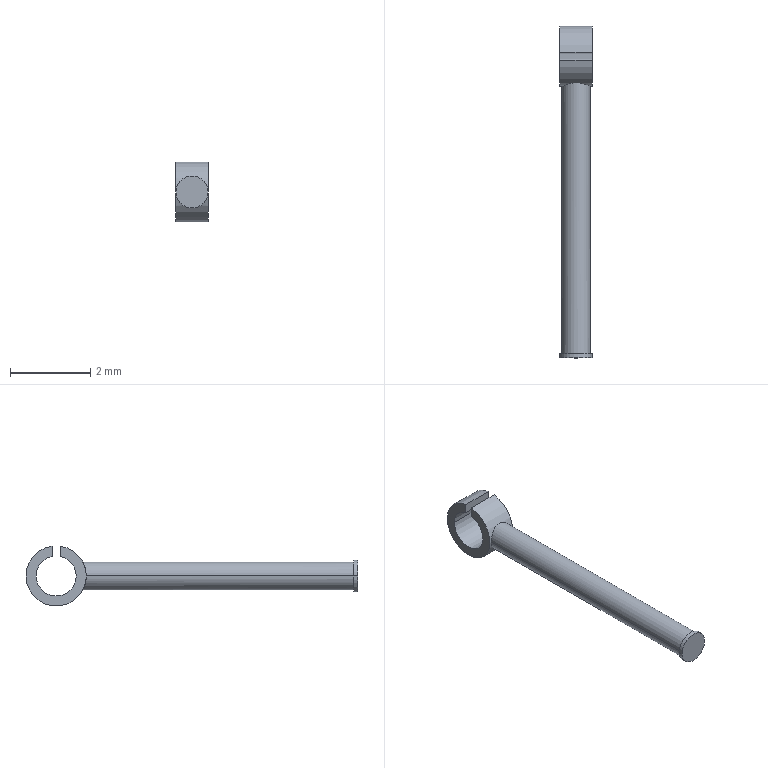Component | SolidWorks | PushRod-15 | 1 solid | 16 faces | box 0.8 x 8.26 x 1.49 mm | volume 3 mm3 | cylinder 10 | plane 6 | commonest cylinder face diameters 1 x3 1.5 x3 0.8 x2 0.7 x2
build123d program:
from build123d import *

# Parameters (mm, degrees)
BOSS_EXTRUDE1_DEPTH      = 3.75
BOSS_EXTRUDE1_DEPTH_BACK = 3
SKETCH2_R                = 0.35
SKETCH3_R                = 0.75
SKETCH3_R_2              = 0.5
BOSS_EXTRUDE2_DEPTH      = 0.4
SKETCH4_R                = 0.4
BOSS_EXTRUDE3_DEPTH      = 0.1
SKETCH5_W                = 0.2
SKETCH5_H                = 0.7342
CUT_EXTRUDE1_DEPTH       = 1


with BuildPart() as part:
    # Sketch2 → Boss-Extrude1 (new, two sides: drawn at the far end of the back side and taken through both)
    with BuildSketch(Plane.XY.offset(-BOSS_EXTRUDE1_DEPTH_BACK)):
        with Locations((-0.5, 1.5)):
            Circle(SKETCH2_R)
    extrude(amount=BOSS_EXTRUDE1_DEPTH + BOSS_EXTRUDE1_DEPTH_BACK)

    # Sketch3 → Boss-Extrude2 (add, symmetric)
    with BuildSketch(Plane(origin=(-0.5, 0, 0), x_dir=(0, 0, -1), z_dir=(1, 0, 0))):
        with Locations((-4.413, 1.5)):
            Circle(SKETCH3_R)
        with Locations((-4.413, 1.5)):
            Circle(SKETCH3_R_2, mode=Mode.SUBTRACT)
    extrude(amount=BOSS_EXTRUDE2_DEPTH, both=True)

    # Sketch4 → Boss-Extrude3 (add)
    with BuildSketch(Plane(origin=(0, 0, -3), x_dir=(-1, 0, 0), z_dir=(0, 0, -1))):
        with Locations((0.5, 1.5)):
            Circle(SKETCH4_R)
    extrude(amount=BOSS_EXTRUDE3_DEPTH)

    # Sketch5 → Cut-Extrude1 (cut)
    with BuildSketch(Plane(origin=(-0.1, 0, 0), x_dir=(0, 0, -1), z_dir=(1, 0, 0))):
        with Locations((-4.413, 0.75)):
            Rectangle(SKETCH5_W, SKETCH5_H)
    extrude(amount=-CUT_EXTRUDE1_DEPTH, mode=Mode.SUBTRACT)


solid = part.part

# Placed as in the assembly
solid = solid.moved(Location((10.347, 3.138, 9), (-90, 0, 0)))
STEP:
#1=COLOUR_RGB('',0.7922,0.8196,0.9333);
#2=FILL_AREA_STYLE_COLOUR('',#1);
#3=FILL_AREA_STYLE('',(#2));
#4=SURFACE_STYLE_FILL_AREA(#3);
#5=SURFACE_SIDE_STYLE('',(#4));
#6=SURFACE_STYLE_USAGE(.BOTH.,#5);
#7=PRESENTATION_STYLE_ASSIGNMENT((#6));
#8=CARTESIAN_POINT('',(0.3719,0.001518,0.2953));
#9=VERTEX_POINT('',#8);
#10=CARTESIAN_POINT('',(0.4034,0.001518,0.2953));
#11=VERTEX_POINT('',#10);
#12=CARTESIAN_POINT('',(0.3877,0.001518,0.2953));
#13=DIRECTION('',(0.,-1.,0.));
#14=DIRECTION('',(-1.,-0.,0.));
#15=AXIS2_PLACEMENT_3D('',#12,#13,#14);
#16=CIRCLE('',#15,0.01575);
#17=EDGE_CURVE('',#9,#11,#16,.T.);
#18=ORIENTED_EDGE('',*,*,#17,.F.);
#19=CARTESIAN_POINT('',(0.3719,0.005455,0.2953));
#20=VERTEX_POINT('',#19);
#21=CARTESIAN_POINT('',(0.3719,0.001518,0.2953));
#22=DIRECTION('',(-0.,1.,-0.));
#23=VECTOR('',#22,39.37);
#24=LINE('',#21,#23);
#25=EDGE_CURVE('',#9,#20,#24,.T.);
#26=ORIENTED_EDGE('',*,*,#25,.T.);
#27=CARTESIAN_POINT('',(0.4034,0.005455,0.2953));
#28=VERTEX_POINT('',#27);
#29=CARTESIAN_POINT('',(0.3877,0.005455,0.2953));
#30=DIRECTION('',(0.,-1.,0.));
#31=DIRECTION('',(-1.,-0.,0.));
#32=AXIS2_PLACEMENT_3D('',#29,#30,#31);
#33=CIRCLE('',#32,0.01575);
#34=EDGE_CURVE('',#20,#28,#33,.T.);
#35=ORIENTED_EDGE('',*,*,#34,.T.);
#36=CARTESIAN_POINT('',(0.4034,0.001518,0.2953));
#37=DIRECTION('',(-0.,1.,-0.));
#38=VECTOR('',#37,39.37);
#39=LINE('',#36,#38);
#40=EDGE_CURVE('',#11,#28,#39,.T.);
#41=ORIENTED_EDGE('',*,*,#40,.F.);
#42=EDGE_LOOP('',(#18,#26,#35,#41));
#43=FACE_OUTER_BOUND('',#42,.T.);
#44=CARTESIAN_POINT('',(0.3877,0.001518,0.2953));
#45=DIRECTION('',(-0.,1.,-0.));
#46=DIRECTION('',(1.,0.,0.));
#47=AXIS2_PLACEMENT_3D('',#44,#45,#46);
#48=CYLINDRICAL_SURFACE('',#47,0.01575);
#49=ADVANCED_FACE('',(#43),#48,.T.);
#50=CARTESIAN_POINT('',(0.4034,0.2934,0.3146));
#51=VERTEX_POINT('',#50);
#52=CARTESIAN_POINT('',(0.4034,0.2776,0.2953));
#53=VERTEX_POINT('',#52);
#54=CARTESIAN_POINT('',(0.4034,0.2973,0.2953));
#55=DIRECTION('',(1.,0.,0.));
#56=DIRECTION('',(0.,-1.,0.));
#57=AXIS2_PLACEMENT_3D('',#54,#55,#56);
#58=CIRCLE('',#57,0.01969);
#59=EDGE_CURVE('',#51,#53,#58,.T.);
#60=ORIENTED_EDGE('',*,*,#59,.T.);
#61=CARTESIAN_POINT('',(0.3719,0.2776,0.2953));
#62=VERTEX_POINT('',#61);
#63=CARTESIAN_POINT('',(0.4034,0.2776,0.2953));
#64=DIRECTION('',(-1.,-0.,0.));
#65=VECTOR('',#64,39.37);
#66=LINE('',#63,#65);
#67=EDGE_CURVE('',#53,#62,#66,.T.);
#68=ORIENTED_EDGE('',*,*,#67,.T.);
#69=CARTESIAN_POINT('',(0.3719,0.2934,0.3146));
#70=VERTEX_POINT('',#69);
#71=CARTESIAN_POINT('',(0.3719,0.2973,0.2953));
#72=DIRECTION('',(1.,0.,0.));
#73=DIRECTION('',(0.,-1.,0.));
#74=AXIS2_PLACEMENT_3D('',#71,#72,#73);
#75=CIRCLE('',#74,0.01969);
#76=EDGE_CURVE('',#70,#62,#75,.T.);
#77=ORIENTED_EDGE('',*,*,#76,.F.);
#78=CARTESIAN_POINT('',(0.4034,0.2934,0.3146));
#79=DIRECTION('',(-1.,-0.,0.));
#80=VECTOR('',#79,39.37);
#81=LINE('',#78,#80);
#82=EDGE_CURVE('',#51,#70,#81,.T.);
#83=ORIENTED_EDGE('',*,*,#82,.F.);
#84=EDGE_LOOP('',(#60,#68,#77,#83));
#85=FACE_OUTER_BOUND('',#84,.T.);
#86=CARTESIAN_POINT('',(0.4034,0.2973,0.2953));
#87=DIRECTION('',(-1.,-0.,0.));
#88=DIRECTION('',(0.,1.,0.));
#89=AXIS2_PLACEMENT_3D('',#86,#87,#88);
#90=CYLINDRICAL_SURFACE('',#89,0.01969);
#91=ADVANCED_FACE('',(#85),#90,.F.);
#92=ORIENTED_EDGE('',*,*,#67,.F.);
#93=CARTESIAN_POINT('',(0.4034,0.317,0.2953));
#94=VERTEX_POINT('',#93);
#95=CARTESIAN_POINT('',(0.4034,0.2973,0.2953));
#96=DIRECTION('',(1.,0.,0.));
#97=DIRECTION('',(0.,-1.,0.));
#98=AXIS2_PLACEMENT_3D('',#95,#96,#97);
#99=CIRCLE('',#98,0.01969);
#100=EDGE_CURVE('',#53,#94,#99,.T.);
#101=ORIENTED_EDGE('',*,*,#100,.T.);
#102=CARTESIAN_POINT('',(0.3719,0.317,0.2953));
#103=VERTEX_POINT('',#102);
#104=CARTESIAN_POINT('',(0.4034,0.317,0.2953));
#105=DIRECTION('',(-1.,-0.,0.));
#106=VECTOR('',#105,39.37);
#107=LINE('',#104,#106);
#108=EDGE_CURVE('',#94,#103,#107,.T.);
#109=ORIENTED_EDGE('',*,*,#108,.T.);
#110=CARTESIAN_POINT('',(0.3719,0.2973,0.2953));
#111=DIRECTION('',(1.,0.,0.));
#112=DIRECTION('',(0.,-1.,0.));
#113=AXIS2_PLACEMENT_3D('',#110,#111,#112);
#114=CIRCLE('',#113,0.01969);
#115=EDGE_CURVE('',#62,#103,#114,.T.);
#116=ORIENTED_EDGE('',*,*,#115,.F.);
#117=EDGE_LOOP('',(#92,#101,#109,#116));
#118=FACE_OUTER_BOUND('',#117,.T.);
#119=CARTESIAN_POINT('',(0.4034,0.2973,0.2953));
#120=DIRECTION('',(-1.,-0.,0.));
#121=DIRECTION('',(0.,1.,0.));
#122=AXIS2_PLACEMENT_3D('',#119,#120,#121);
#123=CYLINDRICAL_SURFACE('',#122,0.01969);
#124=ADVANCED_FACE('',(#118),#123,.F.);
#125=CARTESIAN_POINT('',(0.4034,0.2678,0.2953));
#126=VERTEX_POINT('',#125);
#127=CARTESIAN_POINT('',(0.4034,0.3268,0.2953));
#128=VERTEX_POINT('',#127);
#129=CARTESIAN_POINT('',(0.4034,0.2973,0.2953));
#130=DIRECTION('',(1.,0.,0.));
#131=DIRECTION('',(0.,-1.,0.));
#132=AXIS2_PLACEMENT_3D('',#129,#130,#131);
#133=CIRCLE('',#132,0.02953);
#134=EDGE_CURVE('',#126,#128,#133,.T.);
#135=ORIENTED_EDGE('',*,*,#134,.F.);
#136=CARTESIAN_POINT('',(0.4015,0.2678,0.2953));
#137=VERTEX_POINT('',#136);
#138=CARTESIAN_POINT('',(0.4034,0.2678,0.2953));
#139=DIRECTION('',(-1.,-0.,0.));
#140=VECTOR('',#139,39.37);
#141=LINE('',#138,#140);
#142=EDGE_CURVE('',#126,#137,#141,.T.);
#143=ORIENTED_EDGE('',*,*,#142,.T.);
#144=CARTESIAN_POINT('',(0.3739,0.2678,0.2953));
#145=VERTEX_POINT('',#144);
#146=CARTESIAN_POINT('',(0.4015,0.2678,0.2953));
#147=CARTESIAN_POINT('',(0.4015,0.2678,0.2916));
#148=CARTESIAN_POINT('',(0.3999,0.2686,0.288));
#149=CARTESIAN_POINT('',(0.3949,0.2703,0.283));
#150=CARTESIAN_POINT('',(0.3913,0.2712,0.2815));
#151=CARTESIAN_POINT('',(0.384,0.2712,0.2815));
#152=CARTESIAN_POINT('',(0.3804,0.2703,0.283));
#153=CARTESIAN_POINT('',(0.3754,0.2686,0.2881));
#154=CARTESIAN_POINT('',(0.3739,0.2678,0.2916));
#155=CARTESIAN_POINT('',(0.3739,0.2678,0.2953));
#156=B_SPLINE_CURVE_WITH_KNOTS('',3,(#146,#147,#148,#149,#150,#151,#152,#153,#154,#155),.UNSPECIFIED.,.F.,.F.,(4,2,2,2,4),(0.0005555,0.0008329,0.00111,0.001388,0.001665),.UNSPECIFIED.);
#157=EDGE_CURVE('',#137,#145,#156,.T.);
#158=ORIENTED_EDGE('',*,*,#157,.T.);
#159=CARTESIAN_POINT('',(0.3719,0.2678,0.2953));
#160=VERTEX_POINT('',#159);
#161=CARTESIAN_POINT('',(0.4034,0.2678,0.2953));
#162=DIRECTION('',(-1.,-0.,0.));
#163=VECTOR('',#162,39.37);
#164=LINE('',#161,#163);
#165=EDGE_CURVE('',#145,#160,#164,.T.);
#166=ORIENTED_EDGE('',*,*,#165,.T.);
#167=CARTESIAN_POINT('',(0.3719,0.3268,0.2953));
#168=VERTEX_POINT('',#167);
#169=CARTESIAN_POINT('',(0.3719,0.2973,0.2953));
#170=DIRECTION('',(1.,0.,0.));
#171=DIRECTION('',(0.,-1.,0.));
#172=AXIS2_PLACEMENT_3D('',#169,#170,#171);
#173=CIRCLE('',#172,0.02953);
#174=EDGE_CURVE('',#160,#168,#173,.T.);
#175=ORIENTED_EDGE('',*,*,#174,.T.);
#176=CARTESIAN_POINT('',(0.4034,0.3268,0.2953));
#177=DIRECTION('',(-1.,-0.,0.));
#178=VECTOR('',#177,39.37);
#179=LINE('',#176,#178);
#180=EDGE_CURVE('',#128,#168,#179,.T.);
#181=ORIENTED_EDGE('',*,*,#180,.F.);
#182=EDGE_LOOP('',(#135,#143,#158,#166,#175,#181));
#183=FACE_OUTER_BOUND('',#182,.T.);
#184=CARTESIAN_POINT('',(0.4034,0.2973,0.2953));
#185=DIRECTION('',(-1.,-0.,0.));
#186=DIRECTION('',(0.,1.,0.));
#187=AXIS2_PLACEMENT_3D('',#184,#185,#186);
#188=CYLINDRICAL_SURFACE('',#187,0.02953);
#189=ADVANCED_FACE('',(#183),#188,.T.);
#190=CARTESIAN_POINT('',(0.4034,0.3013,0.3245));
#191=VERTEX_POINT('',#190);
#192=CARTESIAN_POINT('',(0.4034,0.2973,0.2953));
#193=DIRECTION('',(1.,0.,0.));
#194=DIRECTION('',(0.,-1.,0.));
#195=AXIS2_PLACEMENT_3D('',#192,#193,#194);
#196=CIRCLE('',#195,0.02953);
#197=EDGE_CURVE('',#128,#191,#196,.T.);
#198=ORIENTED_EDGE('',*,*,#197,.F.);
#199=ORIENTED_EDGE('',*,*,#180,.T.);
#200=CARTESIAN_POINT('',(0.3719,0.3013,0.3245));
#201=VERTEX_POINT('',#200);
#202=CARTESIAN_POINT('',(0.3719,0.2973,0.2953));
#203=DIRECTION('',(1.,0.,0.));
#204=DIRECTION('',(0.,-1.,0.));
#205=AXIS2_PLACEMENT_3D('',#202,#203,#204);
#206=CIRCLE('',#205,0.02953);
#207=EDGE_CURVE('',#168,#201,#206,.T.);
#208=ORIENTED_EDGE('',*,*,#207,.T.);
#209=CARTESIAN_POINT('',(0.4034,0.3013,0.3245));
#210=DIRECTION('',(1.,0.,0.));
#211=VECTOR('',#210,39.37);
#212=LINE('',#209,#211);
#213=EDGE_CURVE('',#201,#191,#212,.T.);
#214=ORIENTED_EDGE('',*,*,#213,.T.);
#215=EDGE_LOOP('',(#198,#199,#208,#214));
#216=FACE_OUTER_BOUND('',#215,.T.);
#217=CARTESIAN_POINT('',(0.4034,0.2973,0.2953));
#218=DIRECTION('',(-1.,-0.,0.));
#219=DIRECTION('',(0.,1.,0.));
#220=AXIS2_PLACEMENT_3D('',#217,#218,#219);
#221=CYLINDRICAL_SURFACE('',#220,0.02953);
#222=ADVANCED_FACE('',(#216),#221,.T.);
#223=ORIENTED_EDGE('',*,*,#157,.F.);
#224=CARTESIAN_POINT('',(0.4015,0.005455,0.2953));
#225=VERTEX_POINT('',#224);
#226=CARTESIAN_POINT('',(0.4015,0.2712,0.2953));
#227=DIRECTION('',(0.,-1.,0.));
#228=VECTOR('',#227,39.37);
#229=LINE('',#226,#228);
#230=EDGE_CURVE('',#137,#225,#229,.T.);
#231=ORIENTED_EDGE('',*,*,#230,.T.);
#232=CARTESIAN_POINT('',(0.3739,0.005455,0.2953));
#233=VERTEX_POINT('',#232);
#234=CARTESIAN_POINT('',(0.3877,0.005455,0.2953));
#235=DIRECTION('',(-0.,1.,-0.));
#236=DIRECTION('',(1.,0.,0.));
#237=AXIS2_PLACEMENT_3D('',#234,#235,#236);
#238=CIRCLE('',#237,0.01378);
#239=EDGE_CURVE('',#225,#233,#238,.T.);
#240=ORIENTED_EDGE('',*,*,#239,.T.);
#241=CARTESIAN_POINT('',(0.3739,0.2712,0.2953));
#242=DIRECTION('',(0.,-1.,0.));
#243=VECTOR('',#242,39.37);
#244=LINE('',#241,#243);
#245=EDGE_CURVE('',#145,#233,#244,.T.);
#246=ORIENTED_EDGE('',*,*,#245,.F.);
#247=EDGE_LOOP('',(#223,#231,#240,#246));
#248=FACE_OUTER_BOUND('',#247,.T.);
#249=CARTESIAN_POINT('',(0.3877,0.2712,0.2953));
#250=DIRECTION('',(0.,-1.,0.));
#251=DIRECTION('',(-1.,0.,0.));
#252=AXIS2_PLACEMENT_3D('',#249,#250,#251);
#253=CYLINDRICAL_SURFACE('',#252,0.01378);
#254=ADVANCED_FACE('',(#248),#253,.T.);
#255=ORIENTED_EDGE('',*,*,#230,.F.);
#256=CARTESIAN_POINT('',(0.3739,0.2678,0.2953));
#257=CARTESIAN_POINT('',(0.3739,0.2678,0.2989));
#258=CARTESIAN_POINT('',(0.3754,0.2686,0.3025));
#259=CARTESIAN_POINT('',(0.3805,0.2703,0.3076));
#260=CARTESIAN_POINT('',(0.384,0.2712,0.3091));
#261=CARTESIAN_POINT('',(0.3914,0.2712,0.309));
#262=CARTESIAN_POINT('',(0.3949,0.2703,0.3075));
#263=CARTESIAN_POINT('',(0.3999,0.2686,0.3025));
#264=CARTESIAN_POINT('',(0.4015,0.2678,0.2989));
#265=CARTESIAN_POINT('',(0.4015,0.2678,0.2953));
#266=B_SPLINE_CURVE_WITH_KNOTS('',3,(#256,#257,#258,#259,#260,#261,#262,#263,#264,#265),.UNSPECIFIED.,.F.,.F.,(4,2,2,2,4),(0.001665,0.001943,0.00222,0.002498,0.002775),.UNSPECIFIED.);
#267=EDGE_CURVE('',#145,#137,#266,.T.);
#268=ORIENTED_EDGE('',*,*,#267,.F.);
#269=ORIENTED_EDGE('',*,*,#245,.T.);
#270=CARTESIAN_POINT('',(0.3877,0.005455,0.2953));
#271=DIRECTION('',(-0.,1.,-0.));
#272=DIRECTION('',(1.,0.,0.));
#273=AXIS2_PLACEMENT_3D('',#270,#271,#272);
#274=CIRCLE('',#273,0.01378);
#275=EDGE_CURVE('',#233,#225,#274,.T.);
#276=ORIENTED_EDGE('',*,*,#275,.T.);
#277=EDGE_LOOP('',(#255,#268,#269,#276));
#278=FACE_OUTER_BOUND('',#277,.T.);
#279=CARTESIAN_POINT('',(0.3877,0.2712,0.2953));
#280=DIRECTION('',(0.,-1.,0.));
#281=DIRECTION('',(-1.,0.,0.));
#282=AXIS2_PLACEMENT_3D('',#279,#280,#281);
#283=CYLINDRICAL_SURFACE('',#282,0.01378);
#284=ADVANCED_FACE('',(#278),#283,.T.);
#285=ORIENTED_EDGE('',*,*,#142,.F.);
#286=CARTESIAN_POINT('',(0.4034,0.2934,0.3245));
#287=VERTEX_POINT('',#286);
#288=CARTESIAN_POINT('',(0.4034,0.2973,0.2953));
#289=DIRECTION('',(1.,0.,0.));
#290=DIRECTION('',(0.,-1.,0.));
#291=AXIS2_PLACEMENT_3D('',#288,#289,#290);
#292=CIRCLE('',#291,0.02953);
#293=EDGE_CURVE('',#287,#126,#292,.T.);
#294=ORIENTED_EDGE('',*,*,#293,.F.);
#295=CARTESIAN_POINT('',(0.3719,0.2934,0.3245));
#296=VERTEX_POINT('',#295);
#297=CARTESIAN_POINT('',(0.4034,0.2934,0.3245));
#298=DIRECTION('',(-1.,-0.,0.));
#299=VECTOR('',#298,39.37);
#300=LINE('',#297,#299);
#301=EDGE_CURVE('',#287,#296,#300,.T.);
#302=ORIENTED_EDGE('',*,*,#301,.T.);
#303=CARTESIAN_POINT('',(0.3719,0.2973,0.2953));
#304=DIRECTION('',(1.,0.,0.));
#305=DIRECTION('',(0.,-1.,0.));
#306=AXIS2_PLACEMENT_3D('',#303,#304,#305);
#307=CIRCLE('',#306,0.02953);
#308=EDGE_CURVE('',#296,#160,#307,.T.);
#309=ORIENTED_EDGE('',*,*,#308,.T.);
#310=ORIENTED_EDGE('',*,*,#165,.F.);
#311=ORIENTED_EDGE('',*,*,#267,.T.);
#312=EDGE_LOOP('',(#285,#294,#302,#309,#310,#311));
#313=FACE_OUTER_BOUND('',#312,.T.);
#314=CARTESIAN_POINT('',(0.4034,0.2973,0.2953));
#315=DIRECTION('',(-1.,-0.,0.));
#316=DIRECTION('',(0.,1.,0.));
#317=AXIS2_PLACEMENT_3D('',#314,#315,#316);
#318=CYLINDRICAL_SURFACE('',#317,0.02953);
#319=ADVANCED_FACE('',(#313),#318,.T.);
#320=CARTESIAN_POINT('',(0.4034,0.2934,0.3104));
#321=DIRECTION('',(-0.,-0.,-1.));
#322=VECTOR('',#321,39.37);
#323=LINE('',#320,#322);
#324=EDGE_CURVE('',#287,#51,#323,.T.);
#325=ORIENTED_EDGE('',*,*,#324,.F.);
#326=ORIENTED_EDGE('',*,*,#293,.T.);
#327=ORIENTED_EDGE('',*,*,#134,.T.);
#328=ORIENTED_EDGE('',*,*,#197,.T.);
#329=CARTESIAN_POINT('',(0.4034,0.3013,0.3146));
#330=VERTEX_POINT('',#329);
#331=CARTESIAN_POINT('',(0.4034,0.3013,0.3104));
#332=DIRECTION('',(0.,0.,1.));
#333=VECTOR('',#332,39.37);
#334=LINE('',#331,#333);
#335=EDGE_CURVE('',#330,#191,#334,.T.);
#336=ORIENTED_EDGE('',*,*,#335,.F.);
#337=CARTESIAN_POINT('',(0.4034,0.2973,0.2953));
#338=DIRECTION('',(1.,0.,0.));
#339=DIRECTION('',(0.,-1.,0.));
#340=AXIS2_PLACEMENT_3D('',#337,#338,#339);
#341=CIRCLE('',#340,0.01969);
#342=EDGE_CURVE('',#94,#330,#341,.T.);
#343=ORIENTED_EDGE('',*,*,#342,.F.);
#344=ORIENTED_EDGE('',*,*,#100,.F.);
#345=ORIENTED_EDGE('',*,*,#59,.F.);
#346=EDGE_LOOP('',(#325,#326,#327,#328,#336,#343,#344,#345));
#347=FACE_OUTER_BOUND('',#346,.T.);
#348=CARTESIAN_POINT('',(0.4034,0.2973,0.2953));
#349=DIRECTION('',(1.,0.,-0.));
#350=DIRECTION('',(0.,-1.,0.));
#351=AXIS2_PLACEMENT_3D('',#348,#349,#350);
#352=PLANE('',#351);
#353=ADVANCED_FACE('',(#347),#352,.T.);
#354=ORIENTED_EDGE('',*,*,#308,.F.);
#355=CARTESIAN_POINT('',(0.3719,0.2934,0.2953));
#356=DIRECTION('',(-0.,-0.,-1.));
#357=VECTOR('',#356,39.37);
#358=LINE('',#355,#357);
#359=EDGE_CURVE('',#296,#70,#358,.T.);
#360=ORIENTED_EDGE('',*,*,#359,.T.);
#361=ORIENTED_EDGE('',*,*,#76,.T.);
#362=ORIENTED_EDGE('',*,*,#115,.T.);
#363=CARTESIAN_POINT('',(0.3719,0.3013,0.3146));
#364=VERTEX_POINT('',#363);
#365=CARTESIAN_POINT('',(0.3719,0.2973,0.2953));
#366=DIRECTION('',(1.,0.,0.));
#367=DIRECTION('',(0.,-1.,0.));
#368=AXIS2_PLACEMENT_3D('',#365,#366,#367);
#369=CIRCLE('',#368,0.01969);
#370=EDGE_CURVE('',#103,#364,#369,.T.);
#371=ORIENTED_EDGE('',*,*,#370,.T.);
#372=CARTESIAN_POINT('',(0.3719,0.3013,0.2953));
#373=DIRECTION('',(0.,0.,1.));
#374=VECTOR('',#373,39.37);
#375=LINE('',#372,#374);
#376=EDGE_CURVE('',#364,#201,#375,.T.);
#377=ORIENTED_EDGE('',*,*,#376,.T.);
#378=ORIENTED_EDGE('',*,*,#207,.F.);
#379=ORIENTED_EDGE('',*,*,#174,.F.);
#380=EDGE_LOOP('',(#354,#360,#361,#362,#371,#377,#378,#379));
#381=FACE_OUTER_BOUND('',#380,.T.);
#382=CARTESIAN_POINT('',(0.3719,0.2973,0.2953));
#383=DIRECTION('',(1.,0.,-0.));
#384=DIRECTION('',(0.,-1.,0.));
#385=AXIS2_PLACEMENT_3D('',#382,#383,#384);
#386=PLANE('',#385);
#387=ADVANCED_FACE('',(#381),#386,.F.);
#388=ORIENTED_EDGE('',*,*,#108,.F.);
#389=ORIENTED_EDGE('',*,*,#342,.T.);
#390=CARTESIAN_POINT('',(0.4034,0.3013,0.3146));
#391=DIRECTION('',(1.,0.,0.));
#392=VECTOR('',#391,39.37);
#393=LINE('',#390,#392);
#394=EDGE_CURVE('',#364,#330,#393,.T.);
#395=ORIENTED_EDGE('',*,*,#394,.F.);
#396=ORIENTED_EDGE('',*,*,#370,.F.);
#397=EDGE_LOOP('',(#388,#389,#395,#396));
#398=FACE_OUTER_BOUND('',#397,.T.);
#399=CARTESIAN_POINT('',(0.4034,0.2973,0.2953));
#400=DIRECTION('',(-1.,-0.,0.));
#401=DIRECTION('',(0.,1.,0.));
#402=AXIS2_PLACEMENT_3D('',#399,#400,#401);
#403=CYLINDRICAL_SURFACE('',#402,0.01969);
#404=ADVANCED_FACE('',(#398),#403,.F.);
#405=ORIENTED_EDGE('',*,*,#25,.F.);
#406=CARTESIAN_POINT('',(0.3877,0.001518,0.2953));
#407=DIRECTION('',(0.,-1.,0.));
#408=DIRECTION('',(-1.,-0.,0.));
#409=AXIS2_PLACEMENT_3D('',#406,#407,#408);
#410=CIRCLE('',#409,0.01575);
#411=EDGE_CURVE('',#11,#9,#410,.T.);
#412=ORIENTED_EDGE('',*,*,#411,.F.);
#413=ORIENTED_EDGE('',*,*,#40,.T.);
#414=CARTESIAN_POINT('',(0.3877,0.005455,0.2953));
#415=DIRECTION('',(0.,-1.,0.));
#416=DIRECTION('',(-1.,-0.,0.));
#417=AXIS2_PLACEMENT_3D('',#414,#415,#416);
#418=CIRCLE('',#417,0.01575);
#419=EDGE_CURVE('',#28,#20,#418,.T.);
#420=ORIENTED_EDGE('',*,*,#419,.T.);
#421=EDGE_LOOP('',(#405,#412,#413,#420));
#422=FACE_OUTER_BOUND('',#421,.T.);
#423=CARTESIAN_POINT('',(0.3877,0.001518,0.2953));
#424=DIRECTION('',(-0.,1.,-0.));
#425=DIRECTION('',(1.,0.,0.));
#426=AXIS2_PLACEMENT_3D('',#423,#424,#425);
#427=CYLINDRICAL_SURFACE('',#426,0.01575);
#428=ADVANCED_FACE('',(#422),#427,.T.);
#429=ORIENTED_EDGE('',*,*,#411,.T.);
#430=ORIENTED_EDGE('',*,*,#17,.T.);
#431=EDGE_LOOP('',(#429,#430));
#432=FACE_OUTER_BOUND('',#431,.T.);
#433=CARTESIAN_POINT('',(0.3877,0.001518,0.2953));
#434=DIRECTION('',(0.,-1.,0.));
#435=DIRECTION('',(-1.,-0.,0.));
#436=AXIS2_PLACEMENT_3D('',#433,#434,#435);
#437=PLANE('',#436);
#438=ADVANCED_FACE('',(#432),#437,.T.);
#439=ORIENTED_EDGE('',*,*,#275,.F.);
#440=ORIENTED_EDGE('',*,*,#239,.F.);
#441=EDGE_LOOP('',(#439,#440));
#442=FACE_BOUND('',#441,.T.);
#443=ORIENTED_EDGE('',*,*,#419,.F.);
#444=ORIENTED_EDGE('',*,*,#34,.F.);
#445=EDGE_LOOP('',(#443,#444));
#446=FACE_OUTER_BOUND('',#445,.T.);
#447=CARTESIAN_POINT('',(0.3877,0.005455,0.2953));
#448=DIRECTION('',(0.,-1.,0.));
#449=DIRECTION('',(-1.,-0.,0.));
#450=AXIS2_PLACEMENT_3D('',#447,#448,#449);
#451=PLANE('',#450);
#452=ADVANCED_FACE('',(#442,#446),#451,.F.);
#453=ORIENTED_EDGE('',*,*,#376,.F.);
#454=ORIENTED_EDGE('',*,*,#394,.T.);
#455=ORIENTED_EDGE('',*,*,#335,.T.);
#456=ORIENTED_EDGE('',*,*,#213,.F.);
#457=EDGE_LOOP('',(#453,#454,#455,#456));
#458=FACE_OUTER_BOUND('',#457,.T.);
#459=CARTESIAN_POINT('',(0.3641,0.3013,0.3104));
#460=DIRECTION('',(-0.,1.,-0.));
#461=DIRECTION('',(1.,0.,0.));
#462=AXIS2_PLACEMENT_3D('',#459,#460,#461);
#463=PLANE('',#462);
#464=ADVANCED_FACE('',(#458),#463,.F.);
#465=ORIENTED_EDGE('',*,*,#324,.T.);
#466=ORIENTED_EDGE('',*,*,#82,.T.);
#467=ORIENTED_EDGE('',*,*,#359,.F.);
#468=ORIENTED_EDGE('',*,*,#301,.F.);
#469=EDGE_LOOP('',(#465,#466,#467,#468));
#470=FACE_OUTER_BOUND('',#469,.T.);
#471=CARTESIAN_POINT('',(0.3641,0.2934,0.3104));
#472=DIRECTION('',(0.,-1.,0.));
#473=DIRECTION('',(-1.,-0.,0.));
#474=AXIS2_PLACEMENT_3D('',#471,#472,#473);
#475=PLANE('',#474);
#476=ADVANCED_FACE('',(#470),#475,.F.);
#477=CLOSED_SHELL('',(#49,#91,#124,#189,#222,#254,#284,#319,#353,#387,#404,#428,#438,#452,#464,#476));
#478=MANIFOLD_SOLID_BREP('',#477);
#479=STYLED_ITEM('',(#7),#478);
#480=PRESENTATION_LAYER_ASSIGNMENT('','',(#479));
#481=(LENGTH_UNIT()NAMED_UNIT(*)SI_UNIT($,.METRE.));
#482=LENGTH_MEASURE_WITH_UNIT(LENGTH_MEASURE(0.0254),#481);
#483=DIMENSIONAL_EXPONENTS(1.,0.,0.,0.,0.,0.,0.);
#484=(CONVERSION_BASED_UNIT('',#482)LENGTH_UNIT()NAMED_UNIT(#483));
#485=UNCERTAINTY_MEASURE_WITH_UNIT(LENGTH_MEASURE(0.00001),#484,'','');
#486=(NAMED_UNIT(*)PLANE_ANGLE_UNIT()SI_UNIT($,.RADIAN.));
#487=(NAMED_UNIT(*)SI_UNIT($,.STERADIAN.)SOLID_ANGLE_UNIT());
#488=(GEOMETRIC_REPRESENTATION_CONTEXT(3)GLOBAL_UNCERTAINTY_ASSIGNED_CONTEXT((#485))GLOBAL_UNIT_ASSIGNED_CONTEXT((#484,#486,#487))REPRESENTATION_CONTEXT('',''));
#489=MECHANICAL_DESIGN_GEOMETRIC_PRESENTATION_REPRESENTATION('',(#479),#488);
#490=CARTESIAN_POINT('',(0.,0.,0.));
#491=DIRECTION('',(0.,0.,1.));
#492=DIRECTION('',(1.,0.,0.));
#493=AXIS2_PLACEMENT_3D('',#490,#491,#492);
#494=(LENGTH_UNIT()NAMED_UNIT(*)SI_UNIT($,.METRE.));
#495=LENGTH_MEASURE_WITH_UNIT(LENGTH_MEASURE(0.0254),#494);
#496=DIMENSIONAL_EXPONENTS(1.,0.,0.,0.,0.,0.,0.);
#497=(CONVERSION_BASED_UNIT('',#495)LENGTH_UNIT()NAMED_UNIT(#496));
#498=UNCERTAINTY_MEASURE_WITH_UNIT(LENGTH_MEASURE(0.00001),#497,'','');
#499=(NAMED_UNIT(*)PLANE_ANGLE_UNIT()SI_UNIT($,.RADIAN.));
#500=(NAMED_UNIT(*)SI_UNIT($,.STERADIAN.)SOLID_ANGLE_UNIT());
#501=(GEOMETRIC_REPRESENTATION_CONTEXT(3)GLOBAL_UNCERTAINTY_ASSIGNED_CONTEXT((#498))GLOBAL_UNIT_ASSIGNED_CONTEXT((#497,#499,#500))REPRESENTATION_CONTEXT('',''));
#502=ADVANCED_BREP_SHAPE_REPRESENTATION('',(#478,#493),#501);